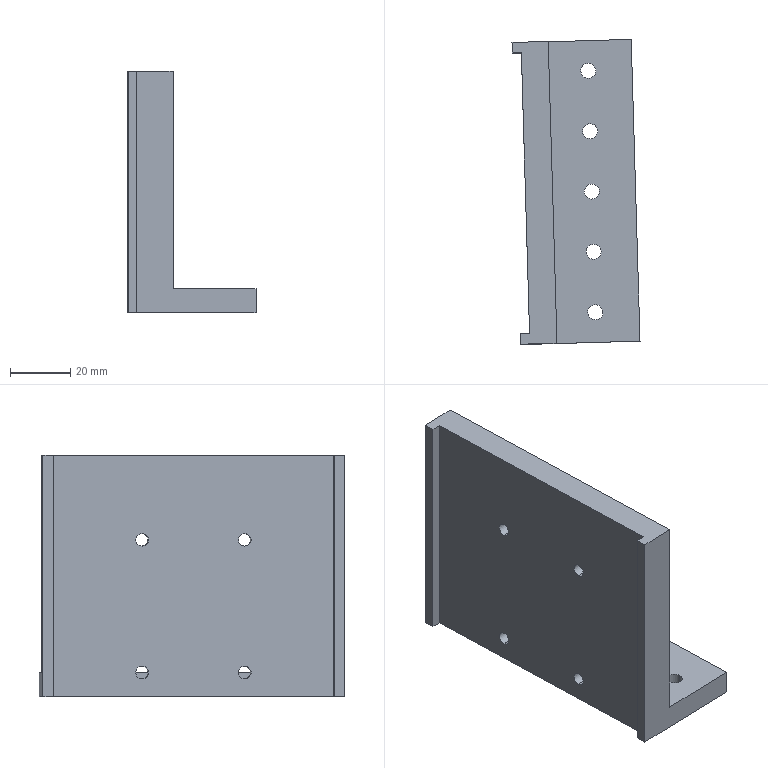Component | SolidWorks | CylinderMountingPlate-1 | 1 solid | 32 faces | box 42.4 x 101.11 x 80 mm | volume 94396 mm3 | cylinder 18 | plane 14 | commonest cylinder face diameters 5 x10 4.2 x8 | material 6063
STEP:
#1=COLOUR_RGB('',0.7922,0.8196,0.9333);
#2=FILL_AREA_STYLE_COLOUR('',#1);
#3=FILL_AREA_STYLE('',(#2));
#4=SURFACE_STYLE_FILL_AREA(#3);
#5=SURFACE_SIDE_STYLE('',(#4));
#6=SURFACE_STYLE_USAGE(.BOTH.,#5);
#7=PRESENTATION_STYLE_ASSIGNMENT((#6));
#8=CARTESIAN_POINT('',(9.938,19.119,-49.378));
#9=VERTEX_POINT('',#8);
#10=CARTESIAN_POINT('',(9.742,19.113,-49.378));
#11=VERTEX_POINT('',#10);
#12=CARTESIAN_POINT('',(9.84,19.116,-49.378));
#13=DIRECTION('',(-0.,0.,-1.));
#14=DIRECTION('',(-0.02918,0.9996,0.));
#15=AXIS2_PLACEMENT_3D('',#12,#13,#14);
#16=CIRCLE('',#15,0.09843);
#17=EDGE_CURVE('',#9,#11,#16,.T.);
#18=ORIENTED_EDGE('',*,*,#17,.F.);
#19=CARTESIAN_POINT('',(9.938,19.119,-49.693));
#20=VERTEX_POINT('',#19);
#21=CARTESIAN_POINT('',(9.938,19.119,-49.693));
#22=DIRECTION('',(-0.,0.,-1.));
#23=VECTOR('',#22,39.37);
#24=LINE('',#21,#23);
#25=EDGE_CURVE('',#9,#20,#24,.T.);
#26=ORIENTED_EDGE('',*,*,#25,.T.);
#27=CARTESIAN_POINT('',(9.742,19.113,-49.693));
#28=VERTEX_POINT('',#27);
#29=CARTESIAN_POINT('',(9.84,19.116,-49.693));
#30=DIRECTION('',(-0.,0.,-1.));
#31=DIRECTION('',(-0.9996,-0.02918,0.));
#32=AXIS2_PLACEMENT_3D('',#29,#30,#31);
#33=CIRCLE('',#32,0.09843);
#34=EDGE_CURVE('',#20,#28,#33,.T.);
#35=ORIENTED_EDGE('',*,*,#34,.T.);
#36=CARTESIAN_POINT('',(9.742,19.113,-49.693));
#37=DIRECTION('',(-0.,0.,-1.));
#38=VECTOR('',#37,39.37);
#39=LINE('',#36,#38);
#40=EDGE_CURVE('',#11,#28,#39,.T.);
#41=ORIENTED_EDGE('',*,*,#40,.F.);
#42=EDGE_LOOP('',(#18,#26,#35,#41));
#43=FACE_OUTER_BOUND('',#42,.T.);
#44=CARTESIAN_POINT('',(9.84,19.116,-49.693));
#45=DIRECTION('',(-0.,0.,-1.));
#46=DIRECTION('',(-0.9996,-0.02918,0.));
#47=AXIS2_PLACEMENT_3D('',#44,#45,#46);
#48=CYLINDRICAL_SURFACE('',#47,0.09843);
#49=ADVANCED_FACE('',(#43),#48,.F.);
#50=CARTESIAN_POINT('',(9.915,19.906,-49.378));
#51=VERTEX_POINT('',#50);
#52=CARTESIAN_POINT('',(9.719,19.9,-49.378));
#53=VERTEX_POINT('',#52);
#54=CARTESIAN_POINT('',(9.817,19.903,-49.378));
#55=DIRECTION('',(-0.,0.,-1.));
#56=DIRECTION('',(-0.02918,0.9996,0.));
#57=AXIS2_PLACEMENT_3D('',#54,#55,#56);
#58=CIRCLE('',#57,0.09843);
#59=EDGE_CURVE('',#51,#53,#58,.T.);
#60=ORIENTED_EDGE('',*,*,#59,.F.);
#61=CARTESIAN_POINT('',(9.915,19.906,-49.693));
#62=VERTEX_POINT('',#61);
#63=CARTESIAN_POINT('',(9.915,19.906,-49.693));
#64=DIRECTION('',(-0.,0.,-1.));
#65=VECTOR('',#64,39.37);
#66=LINE('',#63,#65);
#67=EDGE_CURVE('',#51,#62,#66,.T.);
#68=ORIENTED_EDGE('',*,*,#67,.T.);
#69=CARTESIAN_POINT('',(9.719,19.9,-49.693));
#70=VERTEX_POINT('',#69);
#71=CARTESIAN_POINT('',(9.817,19.903,-49.693));
#72=DIRECTION('',(-0.,0.,-1.));
#73=DIRECTION('',(-0.9996,-0.02918,0.));
#74=AXIS2_PLACEMENT_3D('',#71,#72,#73);
#75=CIRCLE('',#74,0.09843);
#76=EDGE_CURVE('',#62,#70,#75,.T.);
#77=ORIENTED_EDGE('',*,*,#76,.T.);
#78=CARTESIAN_POINT('',(9.719,19.9,-49.693));
#79=DIRECTION('',(-0.,0.,-1.));
#80=VECTOR('',#79,39.37);
#81=LINE('',#78,#80);
#82=EDGE_CURVE('',#53,#70,#81,.T.);
#83=ORIENTED_EDGE('',*,*,#82,.F.);
#84=EDGE_LOOP('',(#60,#68,#77,#83));
#85=FACE_OUTER_BOUND('',#84,.T.);
#86=CARTESIAN_POINT('',(9.817,19.903,-49.693));
#87=DIRECTION('',(-0.,0.,-1.));
#88=DIRECTION('',(-0.9996,-0.02918,0.));
#89=AXIS2_PLACEMENT_3D('',#86,#87,#88);
#90=CYLINDRICAL_SURFACE('',#89,0.09843);
#91=ADVANCED_FACE('',(#85),#90,.F.);
#92=CARTESIAN_POINT('',(9.846,22.267,-49.378));
#93=VERTEX_POINT('',#92);
#94=CARTESIAN_POINT('',(9.65,22.261,-49.378));
#95=VERTEX_POINT('',#94);
#96=CARTESIAN_POINT('',(9.748,22.264,-49.378));
#97=DIRECTION('',(-0.,0.,-1.));
#98=DIRECTION('',(-0.02918,0.9996,0.));
#99=AXIS2_PLACEMENT_3D('',#96,#97,#98);
#100=CIRCLE('',#99,0.09843);
#101=EDGE_CURVE('',#93,#95,#100,.T.);
#102=ORIENTED_EDGE('',*,*,#101,.F.);
#103=CARTESIAN_POINT('',(9.846,22.267,-49.693));
#104=VERTEX_POINT('',#103);
#105=CARTESIAN_POINT('',(9.846,22.267,-49.693));
#106=DIRECTION('',(-0.,0.,-1.));
#107=VECTOR('',#106,39.37);
#108=LINE('',#105,#107);
#109=EDGE_CURVE('',#93,#104,#108,.T.);
#110=ORIENTED_EDGE('',*,*,#109,.T.);
#111=CARTESIAN_POINT('',(9.65,22.261,-49.693));
#112=VERTEX_POINT('',#111);
#113=CARTESIAN_POINT('',(9.748,22.264,-49.693));
#114=DIRECTION('',(-0.,0.,-1.));
#115=DIRECTION('',(-0.9996,-0.02918,0.));
#116=AXIS2_PLACEMENT_3D('',#113,#114,#115);
#117=CIRCLE('',#116,0.09843);
#118=EDGE_CURVE('',#104,#112,#117,.T.);
#119=ORIENTED_EDGE('',*,*,#118,.T.);
#120=CARTESIAN_POINT('',(9.65,22.261,-49.693));
#121=DIRECTION('',(-0.,0.,-1.));
#122=VECTOR('',#121,39.37);
#123=LINE('',#120,#122);
#124=EDGE_CURVE('',#95,#112,#123,.T.);
#125=ORIENTED_EDGE('',*,*,#124,.F.);
#126=EDGE_LOOP('',(#102,#110,#119,#125));
#127=FACE_OUTER_BOUND('',#126,.T.);
#128=CARTESIAN_POINT('',(9.748,22.264,-49.693));
#129=DIRECTION('',(-0.,0.,-1.));
#130=DIRECTION('',(-0.9996,-0.02918,0.));
#131=AXIS2_PLACEMENT_3D('',#128,#129,#130);
#132=CYLINDRICAL_SURFACE('',#131,0.09843);
#133=ADVANCED_FACE('',(#127),#132,.F.);
#134=CARTESIAN_POINT('',(9.869,21.48,-49.378));
#135=VERTEX_POINT('',#134);
#136=CARTESIAN_POINT('',(9.673,21.474,-49.378));
#137=VERTEX_POINT('',#136);
#138=CARTESIAN_POINT('',(9.771,21.477,-49.378));
#139=DIRECTION('',(-0.,0.,-1.));
#140=DIRECTION('',(-0.02918,0.9996,0.));
#141=AXIS2_PLACEMENT_3D('',#138,#139,#140);
#142=CIRCLE('',#141,0.09843);
#143=EDGE_CURVE('',#135,#137,#142,.T.);
#144=ORIENTED_EDGE('',*,*,#143,.F.);
#145=CARTESIAN_POINT('',(9.869,21.48,-49.693));
#146=VERTEX_POINT('',#145);
#147=CARTESIAN_POINT('',(9.869,21.48,-49.693));
#148=DIRECTION('',(-0.,0.,-1.));
#149=VECTOR('',#148,39.37);
#150=LINE('',#147,#149);
#151=EDGE_CURVE('',#135,#146,#150,.T.);
#152=ORIENTED_EDGE('',*,*,#151,.T.);
#153=CARTESIAN_POINT('',(9.673,21.474,-49.693));
#154=VERTEX_POINT('',#153);
#155=CARTESIAN_POINT('',(9.771,21.477,-49.693));
#156=DIRECTION('',(-0.,0.,-1.));
#157=DIRECTION('',(-0.9996,-0.02918,0.));
#158=AXIS2_PLACEMENT_3D('',#155,#156,#157);
#159=CIRCLE('',#158,0.09843);
#160=EDGE_CURVE('',#146,#154,#159,.T.);
#161=ORIENTED_EDGE('',*,*,#160,.T.);
#162=CARTESIAN_POINT('',(9.673,21.474,-49.693));
#163=DIRECTION('',(-0.,0.,-1.));
#164=VECTOR('',#163,39.37);
#165=LINE('',#162,#164);
#166=EDGE_CURVE('',#137,#154,#165,.T.);
#167=ORIENTED_EDGE('',*,*,#166,.F.);
#168=EDGE_LOOP('',(#144,#152,#161,#167));
#169=FACE_OUTER_BOUND('',#168,.T.);
#170=CARTESIAN_POINT('',(9.771,21.477,-49.693));
#171=DIRECTION('',(-0.,0.,-1.));
#172=DIRECTION('',(-0.9996,-0.02918,0.));
#173=AXIS2_PLACEMENT_3D('',#170,#171,#172);
#174=CYLINDRICAL_SURFACE('',#173,0.09843);
#175=ADVANCED_FACE('',(#169),#174,.F.);
#176=CARTESIAN_POINT('',(9.892,20.693,-49.378));
#177=VERTEX_POINT('',#176);
#178=CARTESIAN_POINT('',(9.696,20.687,-49.378));
#179=VERTEX_POINT('',#178);
#180=CARTESIAN_POINT('',(9.794,20.69,-49.378));
#181=DIRECTION('',(-0.,0.,-1.));
#182=DIRECTION('',(-0.02918,0.9996,0.));
#183=AXIS2_PLACEMENT_3D('',#180,#181,#182);
#184=CIRCLE('',#183,0.09843);
#185=EDGE_CURVE('',#177,#179,#184,.T.);
#186=ORIENTED_EDGE('',*,*,#185,.F.);
#187=CARTESIAN_POINT('',(9.892,20.693,-49.693));
#188=VERTEX_POINT('',#187);
#189=CARTESIAN_POINT('',(9.892,20.693,-49.693));
#190=DIRECTION('',(-0.,0.,-1.));
#191=VECTOR('',#190,39.37);
#192=LINE('',#189,#191);
#193=EDGE_CURVE('',#177,#188,#192,.T.);
#194=ORIENTED_EDGE('',*,*,#193,.T.);
#195=CARTESIAN_POINT('',(9.696,20.687,-49.693));
#196=VERTEX_POINT('',#195);
#197=CARTESIAN_POINT('',(9.794,20.69,-49.693));
#198=DIRECTION('',(-0.,0.,-1.));
#199=DIRECTION('',(-0.9996,-0.02918,0.));
#200=AXIS2_PLACEMENT_3D('',#197,#198,#199);
#201=CIRCLE('',#200,0.09843);
#202=EDGE_CURVE('',#188,#196,#201,.T.);
#203=ORIENTED_EDGE('',*,*,#202,.T.);
#204=CARTESIAN_POINT('',(9.696,20.687,-49.693));
#205=DIRECTION('',(-0.,0.,-1.));
#206=VECTOR('',#205,39.37);
#207=LINE('',#204,#206);
#208=EDGE_CURVE('',#179,#196,#207,.T.);
#209=ORIENTED_EDGE('',*,*,#208,.F.);
#210=EDGE_LOOP('',(#186,#194,#203,#209));
#211=FACE_OUTER_BOUND('',#210,.T.);
#212=CARTESIAN_POINT('',(9.794,20.69,-49.693));
#213=DIRECTION('',(-0.,0.,-1.));
#214=DIRECTION('',(-0.9996,-0.02918,0.));
#215=AXIS2_PLACEMENT_3D('',#212,#213,#214);
#216=CYLINDRICAL_SURFACE('',#215,0.09843);
#217=ADVANCED_FACE('',(#211),#216,.F.);
#218=CARTESIAN_POINT('',(8.909,21.334,-47.563));
#219=VERTEX_POINT('',#218);
#220=CARTESIAN_POINT('',(8.909,21.334,-47.729));
#221=VERTEX_POINT('',#220);
#222=CARTESIAN_POINT('',(8.909,21.334,-47.646));
#223=DIRECTION('',(0.9996,0.02918,-0.));
#224=DIRECTION('',(0.,0.,1.));
#225=AXIS2_PLACEMENT_3D('',#222,#223,#224);
#226=CIRCLE('',#225,0.08268);
#227=EDGE_CURVE('',#219,#221,#226,.T.);
#228=ORIENTED_EDGE('',*,*,#227,.F.);
#229=CARTESIAN_POINT('',(9.263,21.344,-47.563));
#230=VERTEX_POINT('',#229);
#231=CARTESIAN_POINT('',(9.263,21.344,-47.563));
#232=DIRECTION('',(0.9996,0.02918,-0.));
#233=VECTOR('',#232,39.37);
#234=LINE('',#231,#233);
#235=EDGE_CURVE('',#219,#230,#234,.T.);
#236=ORIENTED_EDGE('',*,*,#235,.T.);
#237=CARTESIAN_POINT('',(9.263,21.344,-47.729));
#238=VERTEX_POINT('',#237);
#239=CARTESIAN_POINT('',(9.263,21.344,-47.646));
#240=DIRECTION('',(0.9996,0.02918,-0.));
#241=DIRECTION('',(0.,0.,-1.));
#242=AXIS2_PLACEMENT_3D('',#239,#240,#241);
#243=CIRCLE('',#242,0.08268);
#244=EDGE_CURVE('',#230,#238,#243,.T.);
#245=ORIENTED_EDGE('',*,*,#244,.T.);
#246=CARTESIAN_POINT('',(9.263,21.344,-47.729));
#247=DIRECTION('',(0.9996,0.02918,-0.));
#248=VECTOR('',#247,39.37);
#249=LINE('',#246,#248);
#250=EDGE_CURVE('',#221,#238,#249,.T.);
#251=ORIENTED_EDGE('',*,*,#250,.F.);
#252=EDGE_LOOP('',(#228,#236,#245,#251));
#253=FACE_OUTER_BOUND('',#252,.T.);
#254=CARTESIAN_POINT('',(9.263,21.344,-47.646));
#255=DIRECTION('',(0.9996,0.02918,-0.));
#256=DIRECTION('',(0.,0.,-1.));
#257=AXIS2_PLACEMENT_3D('',#254,#255,#256);
#258=CYLINDRICAL_SURFACE('',#257,0.08268);
#259=ADVANCED_FACE('',(#253),#258,.F.);
#260=CARTESIAN_POINT('',(8.909,21.334,-49.296));
#261=VERTEX_POINT('',#260);
#262=CARTESIAN_POINT('',(8.909,21.334,-49.461));
#263=VERTEX_POINT('',#262);
#264=CARTESIAN_POINT('',(8.909,21.334,-49.378));
#265=DIRECTION('',(0.9996,0.02918,-0.));
#266=DIRECTION('',(0.,-0.,1.));
#267=AXIS2_PLACEMENT_3D('',#264,#265,#266);
#268=CIRCLE('',#267,0.08268);
#269=EDGE_CURVE('',#261,#263,#268,.T.);
#270=ORIENTED_EDGE('',*,*,#269,.F.);
#271=CARTESIAN_POINT('',(9.263,21.344,-49.296));
#272=VERTEX_POINT('',#271);
#273=CARTESIAN_POINT('',(9.263,21.344,-49.296));
#274=DIRECTION('',(0.9996,0.02918,-0.));
#275=VECTOR('',#274,39.37);
#276=LINE('',#273,#275);
#277=EDGE_CURVE('',#261,#272,#276,.T.);
#278=ORIENTED_EDGE('',*,*,#277,.T.);
#279=CARTESIAN_POINT('',(9.265,21.261,-49.378));
#280=VERTEX_POINT('',#279);
#281=CARTESIAN_POINT('',(9.263,21.344,-49.378));
#282=DIRECTION('',(0.9996,0.02918,-0.));
#283=DIRECTION('',(0.,0.,-1.));
#284=AXIS2_PLACEMENT_3D('',#281,#282,#283);
#285=CIRCLE('',#284,0.08268);
#286=EDGE_CURVE('',#272,#280,#285,.T.);
#287=ORIENTED_EDGE('',*,*,#286,.T.);
#288=CARTESIAN_POINT('',(9.263,21.344,-49.461));
#289=VERTEX_POINT('',#288);
#290=CARTESIAN_POINT('',(9.263,21.344,-49.378));
#291=DIRECTION('',(0.9996,0.02918,-0.));
#292=DIRECTION('',(0.,0.,-1.));
#293=AXIS2_PLACEMENT_3D('',#290,#291,#292);
#294=CIRCLE('',#293,0.08268);
#295=EDGE_CURVE('',#280,#289,#294,.T.);
#296=ORIENTED_EDGE('',*,*,#295,.T.);
#297=CARTESIAN_POINT('',(9.263,21.344,-49.461));
#298=DIRECTION('',(0.9996,0.02918,-0.));
#299=VECTOR('',#298,39.37);
#300=LINE('',#297,#299);
#301=EDGE_CURVE('',#263,#289,#300,.T.);
#302=ORIENTED_EDGE('',*,*,#301,.F.);
#303=EDGE_LOOP('',(#270,#278,#287,#296,#302));
#304=FACE_OUTER_BOUND('',#303,.T.);
#305=CARTESIAN_POINT('',(9.263,21.344,-49.378));
#306=DIRECTION('',(0.9996,0.02918,-0.));
#307=DIRECTION('',(0.,0.,-1.));
#308=AXIS2_PLACEMENT_3D('',#305,#306,#307);
#309=CYLINDRICAL_SURFACE('',#308,0.08268);
#310=ADVANCED_FACE('',(#304),#309,.F.);
#311=CARTESIAN_POINT('',(8.948,19.996,-49.296));
#312=VERTEX_POINT('',#311);
#313=CARTESIAN_POINT('',(8.948,19.996,-49.461));
#314=VERTEX_POINT('',#313);
#315=CARTESIAN_POINT('',(8.948,19.996,-49.378));
#316=DIRECTION('',(0.9996,0.02918,-0.));
#317=DIRECTION('',(0.,-0.,1.));
#318=AXIS2_PLACEMENT_3D('',#315,#316,#317);
#319=CIRCLE('',#318,0.08268);
#320=EDGE_CURVE('',#312,#314,#319,.T.);
#321=ORIENTED_EDGE('',*,*,#320,.F.);
#322=CARTESIAN_POINT('',(9.302,20.006,-49.296));
#323=VERTEX_POINT('',#322);
#324=CARTESIAN_POINT('',(9.302,20.006,-49.296));
#325=DIRECTION('',(0.9996,0.02918,-0.));
#326=VECTOR('',#325,39.37);
#327=LINE('',#324,#326);
#328=EDGE_CURVE('',#312,#323,#327,.T.);
#329=ORIENTED_EDGE('',*,*,#328,.T.);
#330=CARTESIAN_POINT('',(9.304,19.923,-49.378));
#331=VERTEX_POINT('',#330);
#332=CARTESIAN_POINT('',(9.302,20.006,-49.378));
#333=DIRECTION('',(0.9996,0.02918,-0.));
#334=DIRECTION('',(0.,0.,-1.));
#335=AXIS2_PLACEMENT_3D('',#332,#333,#334);
#336=CIRCLE('',#335,0.08268);
#337=EDGE_CURVE('',#323,#331,#336,.T.);
#338=ORIENTED_EDGE('',*,*,#337,.T.);
#339=CARTESIAN_POINT('',(9.302,20.006,-49.461));
#340=VERTEX_POINT('',#339);
#341=CARTESIAN_POINT('',(9.302,20.006,-49.378));
#342=DIRECTION('',(0.9996,0.02918,-0.));
#343=DIRECTION('',(0.,0.,-1.));
#344=AXIS2_PLACEMENT_3D('',#341,#342,#343);
#345=CIRCLE('',#344,0.08268);
#346=EDGE_CURVE('',#331,#340,#345,.T.);
#347=ORIENTED_EDGE('',*,*,#346,.T.);
#348=CARTESIAN_POINT('',(9.302,20.006,-49.461));
#349=DIRECTION('',(0.9996,0.02918,-0.));
#350=VECTOR('',#349,39.37);
#351=LINE('',#348,#350);
#352=EDGE_CURVE('',#314,#340,#351,.T.);
#353=ORIENTED_EDGE('',*,*,#352,.F.);
#354=EDGE_LOOP('',(#321,#329,#338,#347,#353));
#355=FACE_OUTER_BOUND('',#354,.T.);
#356=CARTESIAN_POINT('',(9.302,20.006,-49.378));
#357=DIRECTION('',(0.9996,0.02918,-0.));
#358=DIRECTION('',(0.,0.,-1.));
#359=AXIS2_PLACEMENT_3D('',#356,#357,#358);
#360=CYLINDRICAL_SURFACE('',#359,0.08268);
#361=ADVANCED_FACE('',(#355),#360,.F.);
#362=CARTESIAN_POINT('',(8.948,19.996,-47.563));
#363=VERTEX_POINT('',#362);
#364=CARTESIAN_POINT('',(8.948,19.996,-47.729));
#365=VERTEX_POINT('',#364);
#366=CARTESIAN_POINT('',(8.948,19.996,-47.646));
#367=DIRECTION('',(0.9996,0.02918,-0.));
#368=DIRECTION('',(0.,-0.,1.));
#369=AXIS2_PLACEMENT_3D('',#366,#367,#368);
#370=CIRCLE('',#369,0.08268);
#371=EDGE_CURVE('',#363,#365,#370,.T.);
#372=ORIENTED_EDGE('',*,*,#371,.F.);
#373=CARTESIAN_POINT('',(9.302,20.006,-47.563));
#374=VERTEX_POINT('',#373);
#375=CARTESIAN_POINT('',(9.302,20.006,-47.563));
#376=DIRECTION('',(0.9996,0.02918,-0.));
#377=VECTOR('',#376,39.37);
#378=LINE('',#375,#377);
#379=EDGE_CURVE('',#363,#374,#378,.T.);
#380=ORIENTED_EDGE('',*,*,#379,.T.);
#381=CARTESIAN_POINT('',(9.302,20.006,-47.729));
#382=VERTEX_POINT('',#381);
#383=CARTESIAN_POINT('',(9.302,20.006,-47.646));
#384=DIRECTION('',(0.9996,0.02918,-0.));
#385=DIRECTION('',(0.,0.,-1.));
#386=AXIS2_PLACEMENT_3D('',#383,#384,#385);
#387=CIRCLE('',#386,0.08268);
#388=EDGE_CURVE('',#374,#382,#387,.T.);
#389=ORIENTED_EDGE('',*,*,#388,.T.);
#390=CARTESIAN_POINT('',(9.302,20.006,-47.729));
#391=DIRECTION('',(0.9996,0.02918,-0.));
#392=VECTOR('',#391,39.37);
#393=LINE('',#390,#392);
#394=EDGE_CURVE('',#365,#382,#393,.T.);
#395=ORIENTED_EDGE('',*,*,#394,.F.);
#396=EDGE_LOOP('',(#372,#380,#389,#395));
#397=FACE_OUTER_BOUND('',#396,.T.);
#398=CARTESIAN_POINT('',(9.302,20.006,-47.646));
#399=DIRECTION('',(0.9996,0.02918,-0.));
#400=DIRECTION('',(0.,0.,-1.));
#401=AXIS2_PLACEMENT_3D('',#398,#399,#400);
#402=CYLINDRICAL_SURFACE('',#401,0.08268);
#403=ADVANCED_FACE('',(#397),#402,.F.);
#404=CARTESIAN_POINT('',(9.84,19.116,-49.693));
#405=DIRECTION('',(-0.,0.,-1.));
#406=DIRECTION('',(-0.9996,-0.02918,0.));
#407=AXIS2_PLACEMENT_3D('',#404,#405,#406);
#408=CIRCLE('',#407,0.09843);
#409=EDGE_CURVE('',#28,#20,#408,.T.);
#410=ORIENTED_EDGE('',*,*,#409,.F.);
#411=ORIENTED_EDGE('',*,*,#34,.F.);
#412=EDGE_LOOP('',(#410,#411));
#413=FACE_BOUND('',#412,.T.);
#414=CARTESIAN_POINT('',(9.817,19.903,-49.693));
#415=DIRECTION('',(-0.,0.,-1.));
#416=DIRECTION('',(-0.9996,-0.02918,0.));
#417=AXIS2_PLACEMENT_3D('',#414,#415,#416);
#418=CIRCLE('',#417,0.09843);
#419=EDGE_CURVE('',#70,#62,#418,.T.);
#420=ORIENTED_EDGE('',*,*,#419,.F.);
#421=ORIENTED_EDGE('',*,*,#76,.F.);
#422=EDGE_LOOP('',(#420,#421));
#423=FACE_BOUND('',#422,.T.);
#424=CARTESIAN_POINT('',(9.748,22.264,-49.693));
#425=DIRECTION('',(-0.,0.,-1.));
#426=DIRECTION('',(-0.9996,-0.02918,0.));
#427=AXIS2_PLACEMENT_3D('',#424,#425,#426);
#428=CIRCLE('',#427,0.09843);
#429=EDGE_CURVE('',#112,#104,#428,.T.);
#430=ORIENTED_EDGE('',*,*,#429,.F.);
#431=ORIENTED_EDGE('',*,*,#118,.F.);
#432=EDGE_LOOP('',(#430,#431));
#433=FACE_BOUND('',#432,.T.);
#434=CARTESIAN_POINT('',(9.771,21.477,-49.693));
#435=DIRECTION('',(-0.,0.,-1.));
#436=DIRECTION('',(-0.9996,-0.02918,0.));
#437=AXIS2_PLACEMENT_3D('',#434,#435,#436);
#438=CIRCLE('',#437,0.09843);
#439=EDGE_CURVE('',#154,#146,#438,.T.);
#440=ORIENTED_EDGE('',*,*,#439,.F.);
#441=ORIENTED_EDGE('',*,*,#160,.F.);
#442=EDGE_LOOP('',(#440,#441));
#443=FACE_BOUND('',#442,.T.);
#444=CARTESIAN_POINT('',(9.794,20.69,-49.693));
#445=DIRECTION('',(-0.,0.,-1.));
#446=DIRECTION('',(-0.9996,-0.02918,0.));
#447=AXIS2_PLACEMENT_3D('',#444,#445,#446);
#448=CIRCLE('',#447,0.09843);
#449=EDGE_CURVE('',#196,#188,#448,.T.);
#450=ORIENTED_EDGE('',*,*,#449,.F.);
#451=ORIENTED_EDGE('',*,*,#202,.F.);
#452=EDGE_LOOP('',(#450,#451));
#453=FACE_BOUND('',#452,.T.);
#454=CARTESIAN_POINT('',(8.875,22.495,-49.693));
#455=VERTEX_POINT('',#454);
#456=CARTESIAN_POINT('',(8.757,22.491,-49.693));
#457=VERTEX_POINT('',#456);
#458=CARTESIAN_POINT('',(8.875,22.495,-49.693));
#459=DIRECTION('',(-0.9996,-0.02918,0.));
#460=VECTOR('',#459,39.37);
#461=LINE('',#458,#460);
#462=EDGE_CURVE('',#455,#457,#461,.T.);
#463=ORIENTED_EDGE('',*,*,#462,.T.);
#464=CARTESIAN_POINT('',(8.753,22.629,-49.693));
#465=VERTEX_POINT('',#464);
#466=CARTESIAN_POINT('',(8.753,22.629,-49.693));
#467=DIRECTION('',(-0.02918,0.9996,0.));
#468=VECTOR('',#467,39.37);
#469=LINE('',#466,#468);
#470=EDGE_CURVE('',#457,#465,#469,.T.);
#471=ORIENTED_EDGE('',*,*,#470,.T.);
#472=CARTESIAN_POINT('',(10.307,22.674,-49.693));
#473=VERTEX_POINT('',#472);
#474=CARTESIAN_POINT('',(9.225,22.643,-49.693));
#475=DIRECTION('',(-0.9996,-0.02918,0.));
#476=VECTOR('',#475,39.37);
#477=LINE('',#474,#476);
#478=EDGE_CURVE('',#473,#465,#477,.T.);
#479=ORIENTED_EDGE('',*,*,#478,.F.);
#480=CARTESIAN_POINT('',(10.422,18.739,-49.693));
#481=VERTEX_POINT('',#480);
#482=CARTESIAN_POINT('',(10.307,22.674,-49.693));
#483=DIRECTION('',(-0.02918,0.9996,0.));
#484=VECTOR('',#483,39.37);
#485=LINE('',#482,#484);
#486=EDGE_CURVE('',#481,#473,#485,.T.);
#487=ORIENTED_EDGE('',*,*,#486,.F.);
#488=CARTESIAN_POINT('',(8.868,18.694,-49.693));
#489=VERTEX_POINT('',#488);
#490=CARTESIAN_POINT('',(9.34,18.707,-49.693));
#491=DIRECTION('',(-0.9996,-0.02918,0.));
#492=VECTOR('',#491,39.37);
#493=LINE('',#490,#492);
#494=EDGE_CURVE('',#481,#489,#493,.T.);
#495=ORIENTED_EDGE('',*,*,#494,.T.);
#496=CARTESIAN_POINT('',(8.864,18.831,-49.693));
#497=VERTEX_POINT('',#496);
#498=CARTESIAN_POINT('',(8.753,22.629,-49.693));
#499=DIRECTION('',(-0.02918,0.9996,0.));
#500=VECTOR('',#499,39.37);
#501=LINE('',#498,#500);
#502=EDGE_CURVE('',#489,#497,#501,.T.);
#503=ORIENTED_EDGE('',*,*,#502,.T.);
#504=CARTESIAN_POINT('',(8.982,18.835,-49.693));
#505=VERTEX_POINT('',#504);
#506=CARTESIAN_POINT('',(8.982,18.835,-49.693));
#507=DIRECTION('',(-0.9996,-0.02918,0.));
#508=VECTOR('',#507,39.37);
#509=LINE('',#506,#508);
#510=EDGE_CURVE('',#505,#497,#509,.T.);
#511=ORIENTED_EDGE('',*,*,#510,.F.);
#512=CARTESIAN_POINT('',(8.982,18.835,-49.693));
#513=DIRECTION('',(-0.02918,0.9996,0.));
#514=VECTOR('',#513,39.37);
#515=LINE('',#512,#514);
#516=EDGE_CURVE('',#505,#455,#515,.T.);
#517=ORIENTED_EDGE('',*,*,#516,.T.);
#518=EDGE_LOOP('',(#463,#471,#479,#487,#495,#503,#511,#517));
#519=FACE_OUTER_BOUND('',#518,.T.);
#520=CARTESIAN_POINT('',(9.225,22.643,-49.693));
#521=DIRECTION('',(0.,-0.,1.));
#522=DIRECTION('',(0.02918,-0.9996,-0.));
#523=AXIS2_PLACEMENT_3D('',#520,#521,#522);
#524=PLANE('',#523);
#525=ADVANCED_FACE('',(#413,#423,#433,#443,#453,#519),#524,.F.);
#526=CARTESIAN_POINT('',(8.875,22.495,-46.544));
#527=VERTEX_POINT('',#526);
#528=CARTESIAN_POINT('',(8.757,22.491,-46.544));
#529=VERTEX_POINT('',#528);
#530=CARTESIAN_POINT('',(8.875,22.495,-46.544));
#531=DIRECTION('',(-0.9996,-0.02918,0.));
#532=VECTOR('',#531,39.37);
#533=LINE('',#530,#532);
#534=EDGE_CURVE('',#527,#529,#533,.T.);
#535=ORIENTED_EDGE('',*,*,#534,.F.);
#536=CARTESIAN_POINT('',(8.982,18.835,-46.544));
#537=VERTEX_POINT('',#536);
#538=CARTESIAN_POINT('',(8.982,18.835,-46.544));
#539=DIRECTION('',(0.02918,-0.9996,-0.));
#540=VECTOR('',#539,39.37);
#541=LINE('',#538,#540);
#542=EDGE_CURVE('',#527,#537,#541,.T.);
#543=ORIENTED_EDGE('',*,*,#542,.T.);
#544=CARTESIAN_POINT('',(8.864,18.831,-46.544));
#545=VERTEX_POINT('',#544);
#546=CARTESIAN_POINT('',(8.982,18.835,-46.544));
#547=DIRECTION('',(-0.9996,-0.02918,0.));
#548=VECTOR('',#547,39.37);
#549=LINE('',#546,#548);
#550=EDGE_CURVE('',#537,#545,#549,.T.);
#551=ORIENTED_EDGE('',*,*,#550,.T.);
#552=CARTESIAN_POINT('',(8.868,18.694,-46.544));
#553=VERTEX_POINT('',#552);
#554=CARTESIAN_POINT('',(8.753,22.629,-46.544));
#555=DIRECTION('',(0.02918,-0.9996,-0.));
#556=VECTOR('',#555,39.37);
#557=LINE('',#554,#556);
#558=EDGE_CURVE('',#545,#553,#557,.T.);
#559=ORIENTED_EDGE('',*,*,#558,.T.);
#560=CARTESIAN_POINT('',(9.34,18.707,-46.544));
#561=VERTEX_POINT('',#560);
#562=CARTESIAN_POINT('',(9.34,18.707,-46.544));
#563=DIRECTION('',(-0.9996,-0.02918,0.));
#564=VECTOR('',#563,39.37);
#565=LINE('',#562,#564);
#566=EDGE_CURVE('',#561,#553,#565,.T.);
#567=ORIENTED_EDGE('',*,*,#566,.F.);
#568=CARTESIAN_POINT('',(9.225,22.643,-46.544));
#569=VERTEX_POINT('',#568);
#570=CARTESIAN_POINT('',(9.225,22.643,-46.544));
#571=DIRECTION('',(0.02918,-0.9996,-0.));
#572=VECTOR('',#571,39.37);
#573=LINE('',#570,#572);
#574=EDGE_CURVE('',#569,#561,#573,.T.);
#575=ORIENTED_EDGE('',*,*,#574,.F.);
#576=CARTESIAN_POINT('',(8.753,22.629,-46.544));
#577=VERTEX_POINT('',#576);
#578=CARTESIAN_POINT('',(9.225,22.643,-46.544));
#579=DIRECTION('',(-0.9996,-0.02918,0.));
#580=VECTOR('',#579,39.37);
#581=LINE('',#578,#580);
#582=EDGE_CURVE('',#569,#577,#581,.T.);
#583=ORIENTED_EDGE('',*,*,#582,.T.);
#584=CARTESIAN_POINT('',(8.753,22.629,-46.544));
#585=DIRECTION('',(0.02918,-0.9996,-0.));
#586=VECTOR('',#585,39.37);
#587=LINE('',#584,#586);
#588=EDGE_CURVE('',#577,#529,#587,.T.);
#589=ORIENTED_EDGE('',*,*,#588,.T.);
#590=EDGE_LOOP('',(#535,#543,#551,#559,#567,#575,#583,#589));
#591=FACE_OUTER_BOUND('',#590,.T.);
#592=CARTESIAN_POINT('',(9.225,22.643,-46.544));
#593=DIRECTION('',(-0.,0.,-1.));
#594=DIRECTION('',(-0.02918,0.9996,0.));
#595=AXIS2_PLACEMENT_3D('',#592,#593,#594);
#596=PLANE('',#595);
#597=ADVANCED_FACE('',(#591),#596,.F.);
#598=CARTESIAN_POINT('',(8.757,22.491,-46.544));
#599=DIRECTION('',(0.,-0.,1.));
#600=VECTOR('',#599,39.37);
#601=LINE('',#598,#600);
#602=EDGE_CURVE('',#457,#529,#601,.T.);
#603=ORIENTED_EDGE('',*,*,#602,.T.);
#604=ORIENTED_EDGE('',*,*,#588,.F.);
#605=CARTESIAN_POINT('',(8.753,22.629,-46.544));
#606=DIRECTION('',(0.,-0.,1.));
#607=VECTOR('',#606,39.37);
#608=LINE('',#605,#607);
#609=EDGE_CURVE('',#465,#577,#608,.T.);
#610=ORIENTED_EDGE('',*,*,#609,.F.);
#611=ORIENTED_EDGE('',*,*,#470,.F.);
#612=EDGE_LOOP('',(#603,#604,#610,#611));
#613=FACE_OUTER_BOUND('',#612,.T.);
#614=CARTESIAN_POINT('',(8.81,20.661,-48.118));
#615=DIRECTION('',(0.9996,0.02918,-0.));
#616=DIRECTION('',(-0.,0.,-1.));
#617=AXIS2_PLACEMENT_3D('',#614,#615,#616);
#618=PLANE('',#617);
#619=ADVANCED_FACE('',(#613),#618,.F.);
#620=CARTESIAN_POINT('',(8.864,18.831,-46.544));
#621=DIRECTION('',(-0.,0.,-1.));
#622=VECTOR('',#621,39.37);
#623=LINE('',#620,#622);
#624=EDGE_CURVE('',#545,#497,#623,.T.);
#625=ORIENTED_EDGE('',*,*,#624,.T.);
#626=ORIENTED_EDGE('',*,*,#502,.F.);
#627=CARTESIAN_POINT('',(8.868,18.694,-46.544));
#628=DIRECTION('',(-0.,0.,-1.));
#629=VECTOR('',#628,39.37);
#630=LINE('',#627,#629);
#631=EDGE_CURVE('',#553,#489,#630,.T.);
#632=ORIENTED_EDGE('',*,*,#631,.F.);
#633=ORIENTED_EDGE('',*,*,#558,.F.);
#634=EDGE_LOOP('',(#625,#626,#632,#633));
#635=FACE_OUTER_BOUND('',#634,.T.);
#636=CARTESIAN_POINT('',(8.81,20.661,-48.118));
#637=DIRECTION('',(0.9996,0.02918,-0.));
#638=DIRECTION('',(-0.,0.,-1.));
#639=AXIS2_PLACEMENT_3D('',#636,#637,#638);
#640=PLANE('',#639);
#641=ADVANCED_FACE('',(#635),#640,.F.);
#642=ORIENTED_EDGE('',*,*,#379,.F.);
#643=CARTESIAN_POINT('',(8.948,19.996,-47.646));
#644=DIRECTION('',(0.9996,0.02918,-0.));
#645=DIRECTION('',(0.,0.,1.));
#646=AXIS2_PLACEMENT_3D('',#643,#644,#645);
#647=CIRCLE('',#646,0.08268);
#648=EDGE_CURVE('',#365,#363,#647,.T.);
#649=ORIENTED_EDGE('',*,*,#648,.F.);
#650=ORIENTED_EDGE('',*,*,#394,.T.);
#651=CARTESIAN_POINT('',(9.302,20.006,-47.646));
#652=DIRECTION('',(0.9996,0.02918,-0.));
#653=DIRECTION('',(0.,0.,-1.));
#654=AXIS2_PLACEMENT_3D('',#651,#652,#653);
#655=CIRCLE('',#654,0.08268);
#656=EDGE_CURVE('',#382,#374,#655,.T.);
#657=ORIENTED_EDGE('',*,*,#656,.T.);
#658=EDGE_LOOP('',(#642,#649,#650,#657));
#659=FACE_OUTER_BOUND('',#658,.T.);
#660=CARTESIAN_POINT('',(9.302,20.006,-47.646));
#661=DIRECTION('',(0.9996,0.02918,-0.));
#662=DIRECTION('',(0.,0.,-1.));
#663=AXIS2_PLACEMENT_3D('',#660,#661,#662);
#664=CYLINDRICAL_SURFACE('',#663,0.08268);
#665=ADVANCED_FACE('',(#659),#664,.F.);
#666=ORIENTED_EDGE('',*,*,#328,.F.);
#667=CARTESIAN_POINT('',(8.948,19.996,-49.378));
#668=DIRECTION('',(0.9996,0.02918,-0.));
#669=DIRECTION('',(0.,0.,1.));
#670=AXIS2_PLACEMENT_3D('',#667,#668,#669);
#671=CIRCLE('',#670,0.08268);
#672=EDGE_CURVE('',#314,#312,#671,.T.);
#673=ORIENTED_EDGE('',*,*,#672,.F.);
#674=ORIENTED_EDGE('',*,*,#352,.T.);
#675=CARTESIAN_POINT('',(9.3,20.089,-49.378));
#676=VERTEX_POINT('',#675);
#677=CARTESIAN_POINT('',(9.302,20.006,-49.378));
#678=DIRECTION('',(0.9996,0.02918,-0.));
#679=DIRECTION('',(0.,0.,-1.));
#680=AXIS2_PLACEMENT_3D('',#677,#678,#679);
#681=CIRCLE('',#680,0.08268);
#682=EDGE_CURVE('',#340,#676,#681,.T.);
#683=ORIENTED_EDGE('',*,*,#682,.T.);
#684=CARTESIAN_POINT('',(9.302,20.006,-49.378));
#685=DIRECTION('',(0.9996,0.02918,-0.));
#686=DIRECTION('',(0.,0.,-1.));
#687=AXIS2_PLACEMENT_3D('',#684,#685,#686);
#688=CIRCLE('',#687,0.08268);
#689=EDGE_CURVE('',#676,#323,#688,.T.);
#690=ORIENTED_EDGE('',*,*,#689,.T.);
#691=EDGE_LOOP('',(#666,#673,#674,#683,#690));
#692=FACE_OUTER_BOUND('',#691,.T.);
#693=CARTESIAN_POINT('',(9.302,20.006,-49.378));
#694=DIRECTION('',(0.9996,0.02918,-0.));
#695=DIRECTION('',(0.,0.,-1.));
#696=AXIS2_PLACEMENT_3D('',#693,#694,#695);
#697=CYLINDRICAL_SURFACE('',#696,0.08268);
#698=ADVANCED_FACE('',(#692),#697,.F.);
#699=ORIENTED_EDGE('',*,*,#277,.F.);
#700=CARTESIAN_POINT('',(8.909,21.334,-49.378));
#701=DIRECTION('',(0.9996,0.02918,-0.));
#702=DIRECTION('',(0.,0.,1.));
#703=AXIS2_PLACEMENT_3D('',#700,#701,#702);
#704=CIRCLE('',#703,0.08268);
#705=EDGE_CURVE('',#263,#261,#704,.T.);
#706=ORIENTED_EDGE('',*,*,#705,.F.);
#707=ORIENTED_EDGE('',*,*,#301,.T.);
#708=CARTESIAN_POINT('',(9.26,21.427,-49.378));
#709=VERTEX_POINT('',#708);
#710=CARTESIAN_POINT('',(9.263,21.344,-49.378));
#711=DIRECTION('',(0.9996,0.02918,-0.));
#712=DIRECTION('',(0.,0.,-1.));
#713=AXIS2_PLACEMENT_3D('',#710,#711,#712);
#714=CIRCLE('',#713,0.08268);
#715=EDGE_CURVE('',#289,#709,#714,.T.);
#716=ORIENTED_EDGE('',*,*,#715,.T.);
#717=CARTESIAN_POINT('',(9.263,21.344,-49.378));
#718=DIRECTION('',(0.9996,0.02918,-0.));
#719=DIRECTION('',(0.,0.,-1.));
#720=AXIS2_PLACEMENT_3D('',#717,#718,#719);
#721=CIRCLE('',#720,0.08268);
#722=EDGE_CURVE('',#709,#272,#721,.T.);
#723=ORIENTED_EDGE('',*,*,#722,.T.);
#724=EDGE_LOOP('',(#699,#706,#707,#716,#723));
#725=FACE_OUTER_BOUND('',#724,.T.);
#726=CARTESIAN_POINT('',(9.263,21.344,-49.378));
#727=DIRECTION('',(0.9996,0.02918,-0.));
#728=DIRECTION('',(0.,0.,-1.));
#729=AXIS2_PLACEMENT_3D('',#726,#727,#728);
#730=CYLINDRICAL_SURFACE('',#729,0.08268);
#731=ADVANCED_FACE('',(#725),#730,.F.);
#732=ORIENTED_EDGE('',*,*,#235,.F.);
#733=CARTESIAN_POINT('',(8.909,21.334,-47.646));
#734=DIRECTION('',(0.9996,0.02918,-0.));
#735=DIRECTION('',(0.,0.,1.));
#736=AXIS2_PLACEMENT_3D('',#733,#734,#735);
#737=CIRCLE('',#736,0.08268);
#738=EDGE_CURVE('',#221,#219,#737,.T.);
#739=ORIENTED_EDGE('',*,*,#738,.F.);
#740=ORIENTED_EDGE('',*,*,#250,.T.);
#741=CARTESIAN_POINT('',(9.263,21.344,-47.646));
#742=DIRECTION('',(0.9996,0.02918,-0.));
#743=DIRECTION('',(0.,0.,-1.));
#744=AXIS2_PLACEMENT_3D('',#741,#742,#743);
#745=CIRCLE('',#744,0.08268);
#746=EDGE_CURVE('',#238,#230,#745,.T.);
#747=ORIENTED_EDGE('',*,*,#746,.T.);
#748=EDGE_LOOP('',(#732,#739,#740,#747));
#749=FACE_OUTER_BOUND('',#748,.T.);
#750=CARTESIAN_POINT('',(9.263,21.344,-47.646));
#751=DIRECTION('',(0.9996,0.02918,-0.));
#752=DIRECTION('',(0.,0.,-1.));
#753=AXIS2_PLACEMENT_3D('',#750,#751,#752);
#754=CYLINDRICAL_SURFACE('',#753,0.08268);
#755=ADVANCED_FACE('',(#749),#754,.F.);
#756=ORIENTED_EDGE('',*,*,#609,.T.);
#757=ORIENTED_EDGE('',*,*,#582,.F.);
#758=CARTESIAN_POINT('',(9.225,22.643,-49.378));
#759=VERTEX_POINT('',#758);
#760=CARTESIAN_POINT('',(9.225,22.643,-46.544));
#761=DIRECTION('',(0.,-0.,1.));
#762=VECTOR('',#761,39.37);
#763=LINE('',#760,#762);
#764=EDGE_CURVE('',#759,#569,#763,.T.);
#765=ORIENTED_EDGE('',*,*,#764,.F.);
#766=CARTESIAN_POINT('',(10.307,22.674,-49.378));
#767=VERTEX_POINT('',#766);
#768=CARTESIAN_POINT('',(10.307,22.674,-49.378));
#769=DIRECTION('',(-0.9996,-0.02918,0.));
#770=VECTOR('',#769,39.37);
#771=LINE('',#768,#770);
#772=EDGE_CURVE('',#767,#759,#771,.T.);
#773=ORIENTED_EDGE('',*,*,#772,.F.);
#774=CARTESIAN_POINT('',(10.307,22.674,-49.693));
#775=DIRECTION('',(0.,-0.,1.));
#776=VECTOR('',#775,39.37);
#777=LINE('',#774,#776);
#778=EDGE_CURVE('',#473,#767,#777,.T.);
#779=ORIENTED_EDGE('',*,*,#778,.F.);
#780=ORIENTED_EDGE('',*,*,#478,.T.);
#781=EDGE_LOOP('',(#756,#757,#765,#773,#779,#780));
#782=FACE_OUTER_BOUND('',#781,.T.);
#783=CARTESIAN_POINT('',(9.225,22.643,-46.544));
#784=DIRECTION('',(0.02918,-0.9996,-0.));
#785=DIRECTION('',(-0.9996,-0.02918,0.));
#786=AXIS2_PLACEMENT_3D('',#783,#784,#785);
#787=PLANE('',#786);
#788=ADVANCED_FACE('',(#782),#787,.F.);
#789=ORIENTED_EDGE('',*,*,#631,.T.);
#790=ORIENTED_EDGE('',*,*,#494,.F.);
#791=CARTESIAN_POINT('',(10.422,18.739,-49.378));
#792=VERTEX_POINT('',#791);
#793=CARTESIAN_POINT('',(10.422,18.739,-49.693));
#794=DIRECTION('',(-0.,0.,-1.));
#795=VECTOR('',#794,39.37);
#796=LINE('',#793,#795);
#797=EDGE_CURVE('',#792,#481,#796,.T.);
#798=ORIENTED_EDGE('',*,*,#797,.F.);
#799=CARTESIAN_POINT('',(9.34,18.707,-49.378));
#800=VERTEX_POINT('',#799);
#801=CARTESIAN_POINT('',(10.422,18.739,-49.378));
#802=DIRECTION('',(-0.9996,-0.02918,0.));
#803=VECTOR('',#802,39.37);
#804=LINE('',#801,#803);
#805=EDGE_CURVE('',#792,#800,#804,.T.);
#806=ORIENTED_EDGE('',*,*,#805,.T.);
#807=CARTESIAN_POINT('',(9.34,18.707,-46.544));
#808=DIRECTION('',(-0.,0.,-1.));
#809=VECTOR('',#808,39.37);
#810=LINE('',#807,#809);
#811=EDGE_CURVE('',#561,#800,#810,.T.);
#812=ORIENTED_EDGE('',*,*,#811,.F.);
#813=ORIENTED_EDGE('',*,*,#566,.T.);
#814=EDGE_LOOP('',(#789,#790,#798,#806,#812,#813));
#815=FACE_OUTER_BOUND('',#814,.T.);
#816=CARTESIAN_POINT('',(9.34,18.707,-46.544));
#817=DIRECTION('',(-0.02918,0.9996,0.));
#818=DIRECTION('',(0.9996,0.02918,-0.));
#819=AXIS2_PLACEMENT_3D('',#816,#817,#818);
#820=PLANE('',#819);
#821=ADVANCED_FACE('',(#815),#820,.F.);
#822=CARTESIAN_POINT('',(9.225,22.643,-49.378));
#823=DIRECTION('',(0.02918,-0.9996,-0.));
#824=VECTOR('',#823,39.37);
#825=LINE('',#822,#824);
#826=EDGE_CURVE('',#759,#709,#825,.T.);
#827=ORIENTED_EDGE('',*,*,#826,.F.);
#828=ORIENTED_EDGE('',*,*,#764,.T.);
#829=ORIENTED_EDGE('',*,*,#574,.T.);
#830=ORIENTED_EDGE('',*,*,#811,.T.);
#831=CARTESIAN_POINT('',(9.225,22.643,-49.378));
#832=DIRECTION('',(0.02918,-0.9996,-0.));
#833=VECTOR('',#832,39.37);
#834=LINE('',#831,#833);
#835=EDGE_CURVE('',#331,#800,#834,.T.);
#836=ORIENTED_EDGE('',*,*,#835,.F.);
#837=ORIENTED_EDGE('',*,*,#337,.F.);
#838=ORIENTED_EDGE('',*,*,#689,.F.);
#839=CARTESIAN_POINT('',(9.225,22.643,-49.378));
#840=DIRECTION('',(0.02918,-0.9996,-0.));
#841=VECTOR('',#840,39.37);
#842=LINE('',#839,#841);
#843=EDGE_CURVE('',#280,#676,#842,.T.);
#844=ORIENTED_EDGE('',*,*,#843,.F.);
#845=ORIENTED_EDGE('',*,*,#286,.F.);
#846=ORIENTED_EDGE('',*,*,#722,.F.);
#847=EDGE_LOOP('',(#827,#828,#829,#830,#836,#837,#838,#844,#845,#846));
#848=FACE_OUTER_BOUND('',#847,.T.);
#849=ORIENTED_EDGE('',*,*,#746,.F.);
#850=ORIENTED_EDGE('',*,*,#244,.F.);
#851=EDGE_LOOP('',(#849,#850));
#852=FACE_BOUND('',#851,.T.);
#853=ORIENTED_EDGE('',*,*,#656,.F.);
#854=ORIENTED_EDGE('',*,*,#388,.F.);
#855=EDGE_LOOP('',(#853,#854));
#856=FACE_BOUND('',#855,.T.);
#857=CARTESIAN_POINT('',(9.282,20.675,-48.118));
#858=DIRECTION('',(0.9996,0.02918,-0.));
#859=DIRECTION('',(-0.,0.,-1.));
#860=AXIS2_PLACEMENT_3D('',#857,#858,#859);
#861=PLANE('',#860);
#862=ADVANCED_FACE('',(#848,#852,#856),#861,.T.);
#863=ORIENTED_EDGE('',*,*,#672,.T.);
#864=ORIENTED_EDGE('',*,*,#320,.T.);
#865=EDGE_LOOP('',(#863,#864));
#866=FACE_BOUND('',#865,.T.);
#867=ORIENTED_EDGE('',*,*,#738,.T.);
#868=ORIENTED_EDGE('',*,*,#227,.T.);
#869=EDGE_LOOP('',(#867,#868));
#870=FACE_BOUND('',#869,.T.);
#871=ORIENTED_EDGE('',*,*,#516,.F.);
#872=CARTESIAN_POINT('',(8.982,18.835,-46.544));
#873=DIRECTION('',(-0.,0.,-1.));
#874=VECTOR('',#873,39.37);
#875=LINE('',#872,#874);
#876=EDGE_CURVE('',#537,#505,#875,.T.);
#877=ORIENTED_EDGE('',*,*,#876,.F.);
#878=ORIENTED_EDGE('',*,*,#542,.F.);
#879=CARTESIAN_POINT('',(8.875,22.495,-46.544));
#880=DIRECTION('',(0.,-0.,1.));
#881=VECTOR('',#880,39.37);
#882=LINE('',#879,#881);
#883=EDGE_CURVE('',#455,#527,#882,.T.);
#884=ORIENTED_EDGE('',*,*,#883,.F.);
#885=EDGE_LOOP('',(#871,#877,#878,#884));
#886=FACE_OUTER_BOUND('',#885,.T.);
#887=ORIENTED_EDGE('',*,*,#705,.T.);
#888=ORIENTED_EDGE('',*,*,#269,.T.);
#889=EDGE_LOOP('',(#887,#888));
#890=FACE_BOUND('',#889,.T.);
#891=ORIENTED_EDGE('',*,*,#648,.T.);
#892=ORIENTED_EDGE('',*,*,#371,.T.);
#893=EDGE_LOOP('',(#891,#892));
#894=FACE_BOUND('',#893,.T.);
#895=CARTESIAN_POINT('',(8.928,20.665,-48.118));
#896=DIRECTION('',(-0.9996,-0.02918,0.));
#897=DIRECTION('',(0.,-0.,1.));
#898=AXIS2_PLACEMENT_3D('',#895,#896,#897);
#899=PLANE('',#898);
#900=ADVANCED_FACE('',(#866,#870,#886,#890,#894),#899,.T.);
#901=ORIENTED_EDGE('',*,*,#602,.F.);
#902=ORIENTED_EDGE('',*,*,#462,.F.);
#903=ORIENTED_EDGE('',*,*,#883,.T.);
#904=ORIENTED_EDGE('',*,*,#534,.T.);
#905=EDGE_LOOP('',(#901,#902,#903,#904));
#906=FACE_OUTER_BOUND('',#905,.T.);
#907=CARTESIAN_POINT('',(8.875,22.495,-46.544));
#908=DIRECTION('',(0.02918,-0.9996,-0.));
#909=DIRECTION('',(-0.9996,-0.02918,0.));
#910=AXIS2_PLACEMENT_3D('',#907,#908,#909);
#911=PLANE('',#910);
#912=ADVANCED_FACE('',(#906),#911,.T.);
#913=ORIENTED_EDGE('',*,*,#624,.F.);
#914=ORIENTED_EDGE('',*,*,#550,.F.);
#915=ORIENTED_EDGE('',*,*,#876,.T.);
#916=ORIENTED_EDGE('',*,*,#510,.T.);
#917=EDGE_LOOP('',(#913,#914,#915,#916));
#918=FACE_OUTER_BOUND('',#917,.T.);
#919=CARTESIAN_POINT('',(8.982,18.835,-46.544));
#920=DIRECTION('',(-0.02918,0.9996,0.));
#921=DIRECTION('',(0.9996,0.02918,-0.));
#922=AXIS2_PLACEMENT_3D('',#919,#920,#921);
#923=PLANE('',#922);
#924=ADVANCED_FACE('',(#918),#923,.T.);
#925=ORIENTED_EDGE('',*,*,#295,.F.);
#926=CARTESIAN_POINT('',(9.225,22.643,-49.378));
#927=DIRECTION('',(0.02918,-0.9996,-0.));
#928=VECTOR('',#927,39.37);
#929=LINE('',#926,#928);
#930=EDGE_CURVE('',#709,#280,#929,.T.);
#931=ORIENTED_EDGE('',*,*,#930,.F.);
#932=ORIENTED_EDGE('',*,*,#715,.F.);
#933=EDGE_LOOP('',(#925,#931,#932));
#934=FACE_OUTER_BOUND('',#933,.T.);
#935=CARTESIAN_POINT('',(9.282,20.675,-48.118));
#936=DIRECTION('',(-0.9996,-0.02918,0.));
#937=DIRECTION('',(0.,-0.,1.));
#938=AXIS2_PLACEMENT_3D('',#935,#936,#937);
#939=PLANE('',#938);
#940=ADVANCED_FACE('',(#934),#939,.T.);
#941=ORIENTED_EDGE('',*,*,#346,.F.);
#942=CARTESIAN_POINT('',(9.225,22.643,-49.378));
#943=DIRECTION('',(0.02918,-0.9996,-0.));
#944=VECTOR('',#943,39.37);
#945=LINE('',#942,#944);
#946=EDGE_CURVE('',#676,#331,#945,.T.);
#947=ORIENTED_EDGE('',*,*,#946,.F.);
#948=ORIENTED_EDGE('',*,*,#682,.F.);
#949=EDGE_LOOP('',(#941,#947,#948));
#950=FACE_OUTER_BOUND('',#949,.T.);
#951=CARTESIAN_POINT('',(9.282,20.675,-48.118));
#952=DIRECTION('',(-0.9996,-0.02918,0.));
#953=DIRECTION('',(0.,-0.,1.));
#954=AXIS2_PLACEMENT_3D('',#951,#952,#953);
#955=PLANE('',#954);
#956=ADVANCED_FACE('',(#950),#955,.T.);
#957=CARTESIAN_POINT('',(9.84,19.116,-49.378));
#958=DIRECTION('',(-0.,0.,-1.));
#959=DIRECTION('',(-0.02918,0.9996,0.));
#960=AXIS2_PLACEMENT_3D('',#957,#958,#959);
#961=CIRCLE('',#960,0.09843);
#962=EDGE_CURVE('',#11,#9,#961,.T.);
#963=ORIENTED_EDGE('',*,*,#962,.T.);
#964=ORIENTED_EDGE('',*,*,#17,.T.);
#965=EDGE_LOOP('',(#963,#964));
#966=FACE_BOUND('',#965,.T.);
#967=CARTESIAN_POINT('',(9.817,19.903,-49.378));
#968=DIRECTION('',(-0.,0.,-1.));
#969=DIRECTION('',(-0.02918,0.9996,0.));
#970=AXIS2_PLACEMENT_3D('',#967,#968,#969);
#971=CIRCLE('',#970,0.09843);
#972=EDGE_CURVE('',#53,#51,#971,.T.);
#973=ORIENTED_EDGE('',*,*,#972,.T.);
#974=ORIENTED_EDGE('',*,*,#59,.T.);
#975=EDGE_LOOP('',(#973,#974));
#976=FACE_BOUND('',#975,.T.);
#977=CARTESIAN_POINT('',(9.748,22.264,-49.378));
#978=DIRECTION('',(-0.,0.,-1.));
#979=DIRECTION('',(-0.02918,0.9996,0.));
#980=AXIS2_PLACEMENT_3D('',#977,#978,#979);
#981=CIRCLE('',#980,0.09843);
#982=EDGE_CURVE('',#95,#93,#981,.T.);
#983=ORIENTED_EDGE('',*,*,#982,.T.);
#984=ORIENTED_EDGE('',*,*,#101,.T.);
#985=EDGE_LOOP('',(#983,#984));
#986=FACE_BOUND('',#985,.T.);
#987=CARTESIAN_POINT('',(9.771,21.477,-49.378));
#988=DIRECTION('',(-0.,0.,-1.));
#989=DIRECTION('',(-0.02918,0.9996,0.));
#990=AXIS2_PLACEMENT_3D('',#987,#988,#989);
#991=CIRCLE('',#990,0.09843);
#992=EDGE_CURVE('',#137,#135,#991,.T.);
#993=ORIENTED_EDGE('',*,*,#992,.T.);
#994=ORIENTED_EDGE('',*,*,#143,.T.);
#995=EDGE_LOOP('',(#993,#994));
#996=FACE_BOUND('',#995,.T.);
#997=CARTESIAN_POINT('',(9.794,20.69,-49.378));
#998=DIRECTION('',(-0.,0.,-1.));
#999=DIRECTION('',(-0.02918,0.9996,0.));
#1000=AXIS2_PLACEMENT_3D('',#997,#998,#999);
#1001=CIRCLE('',#1000,0.09843);
#1002=EDGE_CURVE('',#179,#177,#1001,.T.);
#1003=ORIENTED_EDGE('',*,*,#1002,.T.);
#1004=ORIENTED_EDGE('',*,*,#185,.T.);
#1005=EDGE_LOOP('',(#1003,#1004));
#1006=FACE_BOUND('',#1005,.T.);
#1007=ORIENTED_EDGE('',*,*,#826,.T.);
#1008=ORIENTED_EDGE('',*,*,#930,.T.);
#1009=ORIENTED_EDGE('',*,*,#843,.T.);
#1010=ORIENTED_EDGE('',*,*,#946,.T.);
#1011=ORIENTED_EDGE('',*,*,#835,.T.);
#1012=ORIENTED_EDGE('',*,*,#805,.F.);
#1013=CARTESIAN_POINT('',(10.307,22.674,-49.378));
#1014=DIRECTION('',(0.02918,-0.9996,-0.));
#1015=VECTOR('',#1014,39.37);
#1016=LINE('',#1013,#1015);
#1017=EDGE_CURVE('',#767,#792,#1016,.T.);
#1018=ORIENTED_EDGE('',*,*,#1017,.F.);
#1019=ORIENTED_EDGE('',*,*,#772,.T.);
#1020=EDGE_LOOP('',(#1007,#1008,#1009,#1010,#1011,#1012,#1018,#1019));
#1021=FACE_OUTER_BOUND('',#1020,.T.);
#1022=CARTESIAN_POINT('',(10.307,22.674,-49.378));
#1023=DIRECTION('',(-0.,0.,-1.));
#1024=DIRECTION('',(-0.02918,0.9996,0.));
#1025=AXIS2_PLACEMENT_3D('',#1022,#1023,#1024);
#1026=PLANE('',#1025);
#1027=ADVANCED_FACE('',(#966,#976,#986,#996,#1006,#1021),#1026,.F.);
#1028=ORIENTED_EDGE('',*,*,#486,.T.);
#1029=ORIENTED_EDGE('',*,*,#778,.T.);
#1030=ORIENTED_EDGE('',*,*,#1017,.T.);
#1031=ORIENTED_EDGE('',*,*,#797,.T.);
#1032=EDGE_LOOP('',(#1028,#1029,#1030,#1031));
#1033=FACE_OUTER_BOUND('',#1032,.T.);
#1034=CARTESIAN_POINT('',(10.365,20.707,-48.118));
#1035=DIRECTION('',(-0.9996,-0.02918,0.));
#1036=DIRECTION('',(0.,-0.,1.));
#1037=AXIS2_PLACEMENT_3D('',#1034,#1035,#1036);
#1038=PLANE('',#1037);
#1039=ADVANCED_FACE('',(#1033),#1038,.F.);
#1040=ORIENTED_EDGE('',*,*,#193,.F.);
#1041=ORIENTED_EDGE('',*,*,#1002,.F.);
#1042=ORIENTED_EDGE('',*,*,#208,.T.);
#1043=ORIENTED_EDGE('',*,*,#449,.T.);
#1044=EDGE_LOOP('',(#1040,#1041,#1042,#1043));
#1045=FACE_OUTER_BOUND('',#1044,.T.);
#1046=CARTESIAN_POINT('',(9.794,20.69,-49.693));
#1047=DIRECTION('',(-0.,0.,-1.));
#1048=DIRECTION('',(-0.9996,-0.02918,0.));
#1049=AXIS2_PLACEMENT_3D('',#1046,#1047,#1048);
#1050=CYLINDRICAL_SURFACE('',#1049,0.09843);
#1051=ADVANCED_FACE('',(#1045),#1050,.F.);
#1052=ORIENTED_EDGE('',*,*,#151,.F.);
#1053=ORIENTED_EDGE('',*,*,#992,.F.);
#1054=ORIENTED_EDGE('',*,*,#166,.T.);
#1055=ORIENTED_EDGE('',*,*,#439,.T.);
#1056=EDGE_LOOP('',(#1052,#1053,#1054,#1055));
#1057=FACE_OUTER_BOUND('',#1056,.T.);
#1058=CARTESIAN_POINT('',(9.771,21.477,-49.693));
#1059=DIRECTION('',(-0.,0.,-1.));
#1060=DIRECTION('',(-0.9996,-0.02918,0.));
#1061=AXIS2_PLACEMENT_3D('',#1058,#1059,#1060);
#1062=CYLINDRICAL_SURFACE('',#1061,0.09843);
#1063=ADVANCED_FACE('',(#1057),#1062,.F.);
#1064=ORIENTED_EDGE('',*,*,#109,.F.);
#1065=ORIENTED_EDGE('',*,*,#982,.F.);
#1066=ORIENTED_EDGE('',*,*,#124,.T.);
#1067=ORIENTED_EDGE('',*,*,#429,.T.);
#1068=EDGE_LOOP('',(#1064,#1065,#1066,#1067));
#1069=FACE_OUTER_BOUND('',#1068,.T.);
#1070=CARTESIAN_POINT('',(9.748,22.264,-49.693));
#1071=DIRECTION('',(-0.,0.,-1.));
#1072=DIRECTION('',(-0.9996,-0.02918,0.));
#1073=AXIS2_PLACEMENT_3D('',#1070,#1071,#1072);
#1074=CYLINDRICAL_SURFACE('',#1073,0.09843);
#1075=ADVANCED_FACE('',(#1069),#1074,.F.);
#1076=ORIENTED_EDGE('',*,*,#67,.F.);
#1077=ORIENTED_EDGE('',*,*,#972,.F.);
#1078=ORIENTED_EDGE('',*,*,#82,.T.);
#1079=ORIENTED_EDGE('',*,*,#419,.T.);
#1080=EDGE_LOOP('',(#1076,#1077,#1078,#1079));
#1081=FACE_OUTER_BOUND('',#1080,.T.);
#1082=CARTESIAN_POINT('',(9.817,19.903,-49.693));
#1083=DIRECTION('',(-0.,0.,-1.));
#1084=DIRECTION('',(-0.9996,-0.02918,0.));
#1085=AXIS2_PLACEMENT_3D('',#1082,#1083,#1084);
#1086=CYLINDRICAL_SURFACE('',#1085,0.09843);
#1087=ADVANCED_FACE('',(#1081),#1086,.F.);
#1088=ORIENTED_EDGE('',*,*,#25,.F.);
#1089=ORIENTED_EDGE('',*,*,#962,.F.);
#1090=ORIENTED_EDGE('',*,*,#40,.T.);
#1091=ORIENTED_EDGE('',*,*,#409,.T.);
#1092=EDGE_LOOP('',(#1088,#1089,#1090,#1091));
#1093=FACE_OUTER_BOUND('',#1092,.T.);
#1094=CARTESIAN_POINT('',(9.84,19.116,-49.693));
#1095=DIRECTION('',(-0.,0.,-1.));
#1096=DIRECTION('',(-0.9996,-0.02918,0.));
#1097=AXIS2_PLACEMENT_3D('',#1094,#1095,#1096);
#1098=CYLINDRICAL_SURFACE('',#1097,0.09843);
#1099=ADVANCED_FACE('',(#1093),#1098,.F.);
#1100=CLOSED_SHELL('',(#49,#91,#133,#175,#217,#259,#310,#361,#403,#525,#597,#619,#641,#665,#698,#731,#755,#788,#821,#862,#900,#912,#924,#940,#956,#1027,#1039,#1051,#1063,#1075,#1087,#1099));
#1101=MANIFOLD_SOLID_BREP('',#1100);
#1102=STYLED_ITEM('',(#7),#1101);
#1103=PRESENTATION_LAYER_ASSIGNMENT('','',(#1102));
#1104=CARTESIAN_POINT('',(0.,0.,0.));
#1105=DIRECTION('',(0.,0.,1.));
#1106=DIRECTION('',(1.,0.,0.));
#1107=AXIS2_PLACEMENT_3D('',#1104,#1105,#1106);
#1108=(LENGTH_UNIT()NAMED_UNIT(*)SI_UNIT($,.METRE.));
#1109=LENGTH_MEASURE_WITH_UNIT(LENGTH_MEASURE(0.0254),#1108);
#1110=DIMENSIONAL_EXPONENTS(1.,0.,0.,0.,0.,0.,0.);
#1111=(CONVERSION_BASED_UNIT('',#1109)LENGTH_UNIT()NAMED_UNIT(#1110));
#1112=UNCERTAINTY_MEASURE_WITH_UNIT(LENGTH_MEASURE(0.00001),#1111,'','');
#1113=(NAMED_UNIT(*)PLANE_ANGLE_UNIT()SI_UNIT($,.RADIAN.));
#1114=(NAMED_UNIT(*)SI_UNIT($,.STERADIAN.)SOLID_ANGLE_UNIT());
#1115=(GEOMETRIC_REPRESENTATION_CONTEXT(3)GLOBAL_UNCERTAINTY_ASSIGNED_CONTEXT((#1112))GLOBAL_UNIT_ASSIGNED_CONTEXT((#1111,#1113,#1114))REPRESENTATION_CONTEXT('',''));
#1116=ADVANCED_BREP_SHAPE_REPRESENTATION('',(#1101,#1107),#1115);
#1117=(LENGTH_UNIT()NAMED_UNIT(*)SI_UNIT($,.METRE.));
#1118=LENGTH_MEASURE_WITH_UNIT(LENGTH_MEASURE(0.0254),#1117);
#1119=DIMENSIONAL_EXPONENTS(1.,0.,0.,0.,0.,0.,0.);
#1120=(CONVERSION_BASED_UNIT('',#1118)LENGTH_UNIT()NAMED_UNIT(#1119));
#1121=UNCERTAINTY_MEASURE_WITH_UNIT(LENGTH_MEASURE(0.00001),#1120,'','');
#1122=(NAMED_UNIT(*)PLANE_ANGLE_UNIT()SI_UNIT($,.RADIAN.));
#1123=(NAMED_UNIT(*)SI_UNIT($,.STERADIAN.)SOLID_ANGLE_UNIT());
#1124=(GEOMETRIC_REPRESENTATION_CONTEXT(3)GLOBAL_UNCERTAINTY_ASSIGNED_CONTEXT((#1121))GLOBAL_UNIT_ASSIGNED_CONTEXT((#1120,#1122,#1123))REPRESENTATION_CONTEXT('',''));
#1125=MECHANICAL_DESIGN_GEOMETRIC_PRESENTATION_REPRESENTATION('',(#1102),#1124);